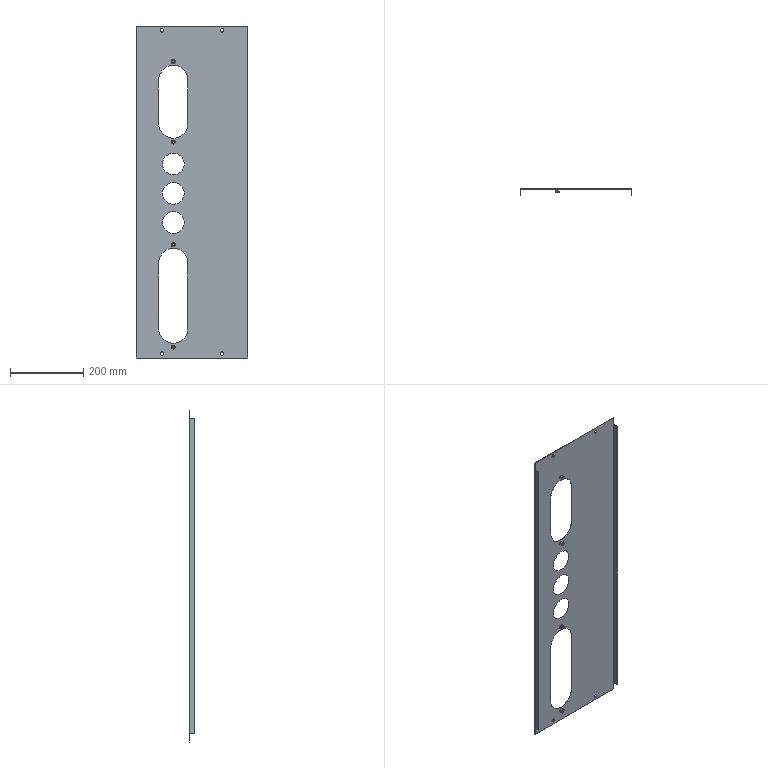Component | SolidWorks | BottomPlateMountingPlate1-1 | 1 solid | 104 faces | volume 308842 mm3 | cylinder 62 | plane 38 | spline 4 | commonest cylinder face diameters 7 x12 3 x10 6 x8 11 x8 8 x8 80 x6 60 x6 0.2 x2